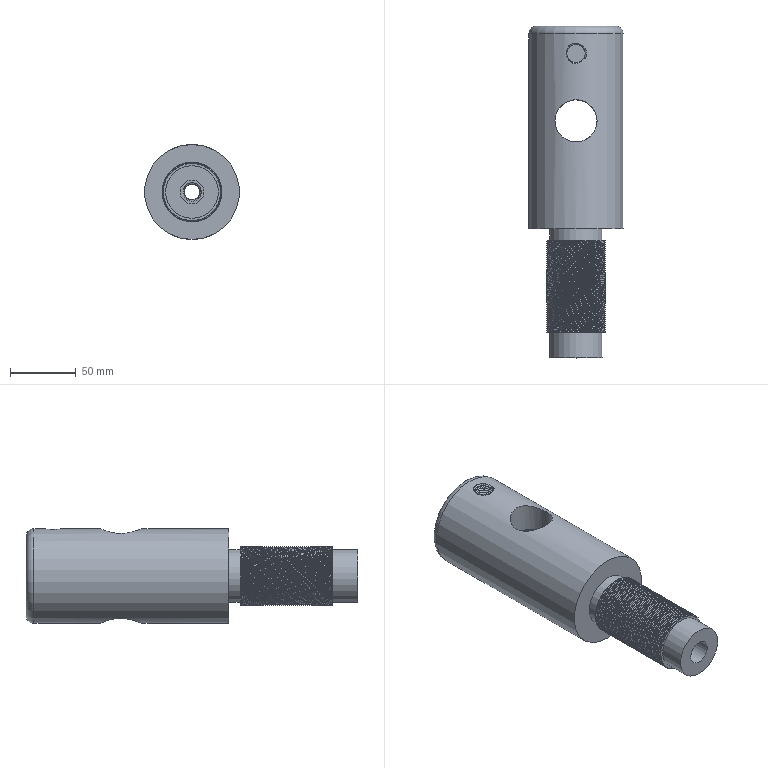Component | NX | TOOL_HOLDER | 1 solid | 32 faces | volume 629944 mm3 | cylinder 12 | plane 10 | spline 9 | torus 1 | commonest cylinder face diameters 14 x3 40 x2 12 x1 72 x1 45 x1 18 x1 32 x1 16 x1